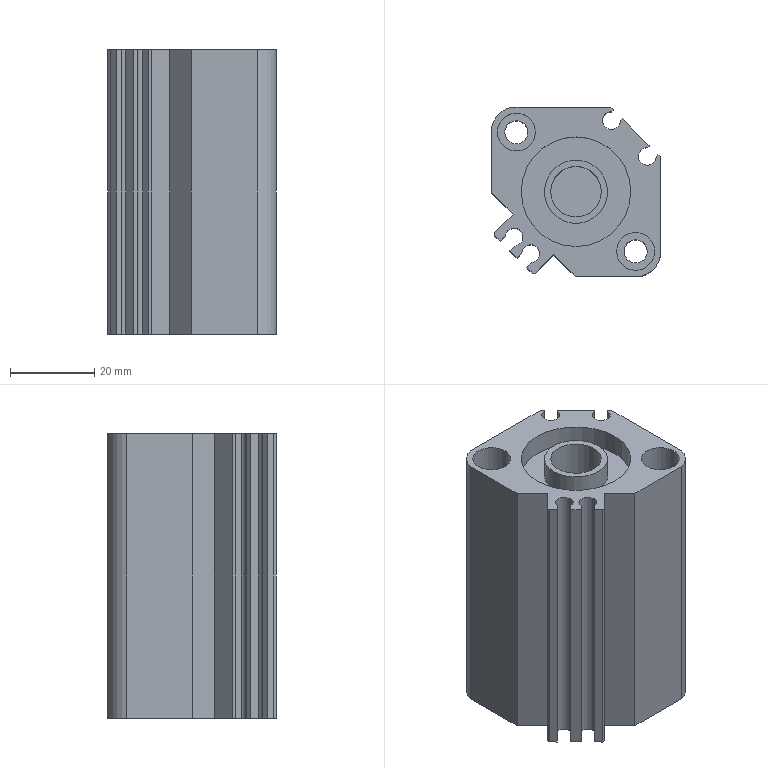Component | SolidWorks | CDQ2B25-35DZ-M9BL-1_CDQ2B25-35-M9B(0_0)_BODY-1 | 1 solid | 79 faces | volume 62980 mm3 | cylinder 38 | plane 37 | cone 4 | commonest cylinder face diameters 4.26 x10 9 x8 5.5 x4 4.134 x4 12 x4 26 x4 25 x2 15 x2